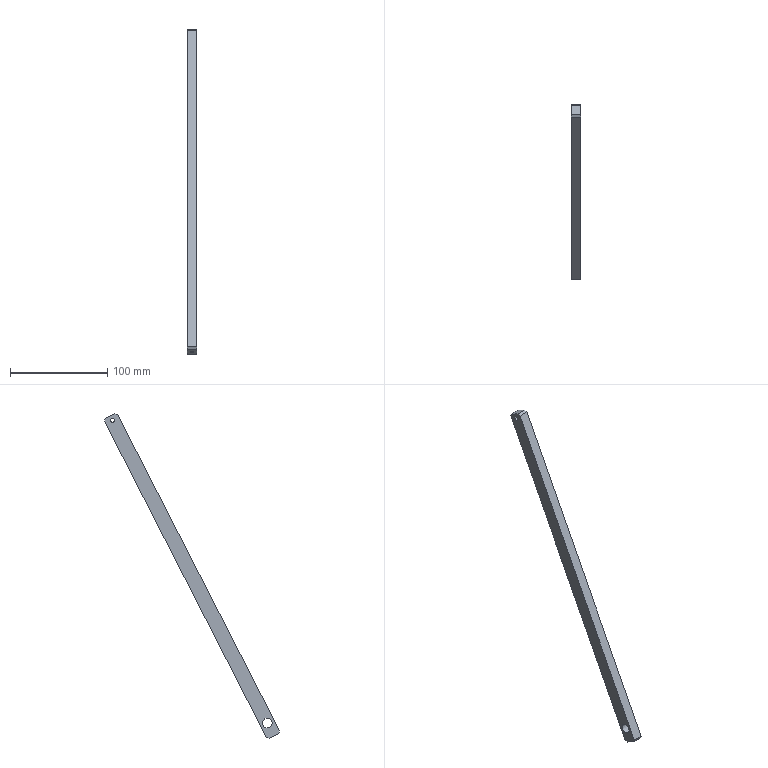Component | SolidWorks | ElectricalBoxAssembly2-1_SwingArm-1 | 1 solid | 16 faces | box 10 x 180.09 x 334.39 mm | volume 54356 mm3 | plane 10 | cylinder 6 | commonest cylinder face diameters 4.2 x4 10 x2
build123d program:
from build123d import *

# Parameters (mm, degrees)
SKETCH1_W             = 370
SKETCH1_H             = 15
SKETCH1_R             = 5
BOSS_EXTRUDE1_DEPTH   = 10
M5_TAPPED_HOLE1_D     = 4.2
M5_TAPPED_HOLE2_D     = 4.2
M5_TAPPED_HOLE2_DEPTH = 15
M5_TAPPED_HOLE2_TIP   = 1.262
CHAMFER1_SIZE         = 2


with BuildPart() as part:
    # Sketch1 → Boss-Extrude1 (new body)
    with BuildSketch(Plane.XY):
        Rectangle(SKETCH1_W, SKETCH1_H)
        with Locations((170, 0)):
            Circle(SKETCH1_R, mode=Mode.SUBTRACT)
    extrude(amount=BOSS_EXTRUDE1_DEPTH)

    # M5 Tapped Hole1 (through all)
    with Locations(Plane.XY.offset(10)):
        with Locations((-180, 0)):
            Hole(M5_TAPPED_HOLE1_D / 2)

    # M5 Tapped Hole2
    with Locations(Plane(origin=(185, 0, 0), x_dir=(0, 0, -1), z_dir=(1, 0, 0))):
        with Locations((-5, 0)):
            Hole(M5_TAPPED_HOLE2_D / 2, depth=M5_TAPPED_HOLE2_DEPTH)
            with Locations((0, 0, -(M5_TAPPED_HOLE2_DEPTH + M5_TAPPED_HOLE2_TIP / 2))):  # 118° drill point
                Cone(0, M5_TAPPED_HOLE2_D / 2, M5_TAPPED_HOLE2_TIP, mode=Mode.SUBTRACT)

    # Chamfer1
    chamfer1_edges = [part.edges().sort_by_distance(p)[0] for p in [
        (185, -7.5, 5),
        (-185, -7.5, 5),
        (-185, 7.5, 5),
        (185, 7.5, 5),
    ]]
    chamfer(chamfer1_edges, length=CHAMFER1_SIZE)


solid = part.part

# Placed as in the assembly
solid = solid.moved(Location((750.468, 292.11, 1827.734), (152.899, -90, 0)))
STEP:
#1=CARTESIAN_POINT('',(29.432,8.362,65.825));
#2=VERTEX_POINT('',#1);
#3=CARTESIAN_POINT('',(29.266,8.362,65.825));
#4=VERTEX_POINT('',#3);
#5=CARTESIAN_POINT('',(29.432,8.362,65.825));
#6=CARTESIAN_POINT('',(29.432,8.367,65.822));
#7=CARTESIAN_POINT('',(29.431,8.372,65.82));
#8=CARTESIAN_POINT('',(29.429,8.381,65.816));
#9=CARTESIAN_POINT('',(29.428,8.386,65.814));
#10=CARTESIAN_POINT('',(29.423,8.396,65.811));
#11=CARTESIAN_POINT('',(29.421,8.401,65.81));
#12=CARTESIAN_POINT('',(29.415,8.41,65.808));
#13=CARTESIAN_POINT('',(29.411,8.414,65.807));
#14=CARTESIAN_POINT('',(29.4,8.426,65.805));
#15=CARTESIAN_POINT('',(29.391,8.432,65.804));
#16=CARTESIAN_POINT('',(29.376,8.439,65.803));
#17=CARTESIAN_POINT('',(29.371,8.441,65.803));
#18=CARTESIAN_POINT('',(29.36,8.443,65.803));
#19=CARTESIAN_POINT('',(29.355,8.444,65.803));
#20=CARTESIAN_POINT('',(29.344,8.444,65.803));
#21=CARTESIAN_POINT('',(29.338,8.443,65.803));
#22=CARTESIAN_POINT('',(29.328,8.441,65.803));
#23=CARTESIAN_POINT('',(29.322,8.439,65.803));
#24=CARTESIAN_POINT('',(29.312,8.434,65.804));
#25=CARTESIAN_POINT('',(29.308,8.432,65.804));
#26=CARTESIAN_POINT('',(29.299,8.425,65.805));
#27=CARTESIAN_POINT('',(29.294,8.422,65.805));
#28=CARTESIAN_POINT('',(29.287,8.414,65.807));
#29=CARTESIAN_POINT('',(29.284,8.41,65.808));
#30=CARTESIAN_POINT('',(29.278,8.401,65.81));
#31=CARTESIAN_POINT('',(29.275,8.396,65.811));
#32=CARTESIAN_POINT('',(29.269,8.382,65.816));
#33=CARTESIAN_POINT('',(29.266,8.371,65.82));
#34=CARTESIAN_POINT('',(29.266,8.362,65.825));
#35=B_SPLINE_CURVE_WITH_KNOTS('',3,(#5,#6,#7,#8,#9,#10,#11,#12,#13,#14,#15,#16,#17,#18,#19,#20,#21,#22,#23,#24,#25,#26,#27,#28,#29,#30,#31,#32,#33,#34),.UNSPECIFIED.,.F.,.F.,(4,2,2,2,2,2,2,2,2,2,2,2,2,2,4),(0.,0.0004152,0.0008304,0.001246,0.001661,0.002491,0.002907,0.003322,0.003737,0.004152,0.004567,0.004983,0.005398,0.005813,0.006644),.UNSPECIFIED.);
#36=EDGE_CURVE('',#2,#4,#35,.T.);
#37=ORIENTED_EDGE('',*,*,#36,.T.);
#38=CARTESIAN_POINT('',(29.266,8.182,65.474));
#39=VERTEX_POINT('',#38);
#40=CARTESIAN_POINT('',(29.266,8.182,65.474));
#41=DIRECTION('',(0.,-0.4556,-0.8902));
#42=VECTOR('',#41,39.37);
#43=LINE('',#40,#42);
#44=EDGE_CURVE('',#4,#39,#43,.T.);
#45=ORIENTED_EDGE('',*,*,#44,.T.);
#46=CARTESIAN_POINT('',(29.432,8.182,65.474));
#47=VERTEX_POINT('',#46);
#48=CARTESIAN_POINT('',(29.349,8.182,65.474));
#49=DIRECTION('',(0.,-0.4556,-0.8902));
#50=DIRECTION('',(1.,0.,0.));
#51=AXIS2_PLACEMENT_3D('',#48,#49,#50);
#52=CIRCLE('',#51,0.08268);
#53=EDGE_CURVE('',#39,#47,#52,.T.);
#54=ORIENTED_EDGE('',*,*,#53,.T.);
#55=CARTESIAN_POINT('',(29.432,8.182,65.474));
#56=DIRECTION('',(0.,-0.4556,-0.8902));
#57=VECTOR('',#56,39.37);
#58=LINE('',#55,#57);
#59=EDGE_CURVE('',#2,#47,#58,.T.);
#60=ORIENTED_EDGE('',*,*,#59,.F.);
#61=EDGE_LOOP('',(#37,#45,#54,#60));
#62=FACE_OUTER_BOUND('',#61,.T.);
#63=CARTESIAN_POINT('',(29.349,8.182,65.474));
#64=DIRECTION('',(0.,-0.4556,-0.8902));
#65=DIRECTION('',(1.,0.,0.));
#66=AXIS2_PLACEMENT_3D('',#63,#64,#65);
#67=CYLINDRICAL_SURFACE('',#66,0.08268);
#68=ADVANCED_FACE('',(#62),#67,.F.);
#69=CARTESIAN_POINT('',(29.546,14.766,78.34));
#70=VERTEX_POINT('',#69);
#71=CARTESIAN_POINT('',(29.546,14.691,78.193));
#72=VERTEX_POINT('',#71);
#73=CARTESIAN_POINT('',(29.546,14.729,78.267));
#74=DIRECTION('',(-1.,0.,-0.));
#75=DIRECTION('',(0.,-0.4556,-0.8902));
#76=AXIS2_PLACEMENT_3D('',#73,#74,#75);
#77=CIRCLE('',#76,0.08268);
#78=EDGE_CURVE('',#70,#72,#77,.T.);
#79=ORIENTED_EDGE('',*,*,#78,.F.);
#80=CARTESIAN_POINT('',(29.152,14.766,78.34));
#81=VERTEX_POINT('',#80);
#82=CARTESIAN_POINT('',(29.152,14.766,78.34));
#83=DIRECTION('',(-1.,0.,-0.));
#84=VECTOR('',#83,39.37);
#85=LINE('',#82,#84);
#86=EDGE_CURVE('',#70,#81,#85,.T.);
#87=ORIENTED_EDGE('',*,*,#86,.T.);
#88=CARTESIAN_POINT('',(29.152,14.691,78.193));
#89=VERTEX_POINT('',#88);
#90=CARTESIAN_POINT('',(29.152,14.729,78.267));
#91=DIRECTION('',(-1.,0.,-0.));
#92=DIRECTION('',(0.,-0.4556,-0.8902));
#93=AXIS2_PLACEMENT_3D('',#90,#91,#92);
#94=CIRCLE('',#93,0.08268);
#95=EDGE_CURVE('',#81,#89,#94,.T.);
#96=ORIENTED_EDGE('',*,*,#95,.T.);
#97=CARTESIAN_POINT('',(29.152,14.691,78.193));
#98=DIRECTION('',(-1.,0.,-0.));
#99=VECTOR('',#98,39.37);
#100=LINE('',#97,#99);
#101=EDGE_CURVE('',#72,#89,#100,.T.);
#102=ORIENTED_EDGE('',*,*,#101,.F.);
#103=EDGE_LOOP('',(#79,#87,#96,#102));
#104=FACE_OUTER_BOUND('',#103,.T.);
#105=CARTESIAN_POINT('',(29.152,14.729,78.267));
#106=DIRECTION('',(-1.,0.,-0.));
#107=DIRECTION('',(0.,-0.4556,-0.8902));
#108=AXIS2_PLACEMENT_3D('',#105,#106,#107);
#109=CYLINDRICAL_SURFACE('',#108,0.08268);
#110=ADVANCED_FACE('',(#104),#109,.F.);
#111=CARTESIAN_POINT('',(29.152,8.541,66.175));
#112=VERTEX_POINT('',#111);
#113=CARTESIAN_POINT('',(29.152,8.362,65.825));
#114=VERTEX_POINT('',#113);
#115=CARTESIAN_POINT('',(29.152,8.451,66.));
#116=DIRECTION('',(-1.,0.,-0.));
#117=DIRECTION('',(0.,-0.4556,-0.8902));
#118=AXIS2_PLACEMENT_3D('',#115,#116,#117);
#119=CIRCLE('',#118,0.1969);
#120=EDGE_CURVE('',#112,#114,#119,.T.);
#121=ORIENTED_EDGE('',*,*,#120,.T.);
#122=CARTESIAN_POINT('',(29.152,8.362,65.825));
#123=DIRECTION('',(1.,0.,0.));
#124=VECTOR('',#123,39.37);
#125=LINE('',#122,#124);
#126=EDGE_CURVE('',#114,#4,#125,.T.);
#127=ORIENTED_EDGE('',*,*,#126,.T.);
#128=ORIENTED_EDGE('',*,*,#36,.F.);
#129=CARTESIAN_POINT('',(29.546,8.362,65.825));
#130=VERTEX_POINT('',#129);
#131=CARTESIAN_POINT('',(29.152,8.362,65.825));
#132=DIRECTION('',(1.,0.,0.));
#133=VECTOR('',#132,39.37);
#134=LINE('',#131,#133);
#135=EDGE_CURVE('',#2,#130,#134,.T.);
#136=ORIENTED_EDGE('',*,*,#135,.T.);
#137=CARTESIAN_POINT('',(29.546,8.541,66.175));
#138=VERTEX_POINT('',#137);
#139=CARTESIAN_POINT('',(29.546,8.451,66.));
#140=DIRECTION('',(-1.,0.,-0.));
#141=DIRECTION('',(0.,-0.4556,-0.8902));
#142=AXIS2_PLACEMENT_3D('',#139,#140,#141);
#143=CIRCLE('',#142,0.1969);
#144=EDGE_CURVE('',#138,#130,#143,.T.);
#145=ORIENTED_EDGE('',*,*,#144,.F.);
#146=CARTESIAN_POINT('',(29.152,8.541,66.175));
#147=DIRECTION('',(1.,0.,0.));
#148=VECTOR('',#147,39.37);
#149=LINE('',#146,#148);
#150=EDGE_CURVE('',#112,#138,#149,.T.);
#151=ORIENTED_EDGE('',*,*,#150,.F.);
#152=EDGE_LOOP('',(#121,#127,#128,#136,#145,#151));
#153=FACE_OUTER_BOUND('',#152,.T.);
#154=CARTESIAN_POINT('',(29.152,8.451,66.));
#155=DIRECTION('',(1.,0.,0.));
#156=DIRECTION('',(0.,0.4556,0.8902));
#157=AXIS2_PLACEMENT_3D('',#154,#155,#156);
#158=CYLINDRICAL_SURFACE('',#157,0.1969);
#159=ADVANCED_FACE('',(#153),#158,.F.);
#160=CARTESIAN_POINT('',(29.152,14.729,78.267));
#161=DIRECTION('',(-1.,0.,-0.));
#162=DIRECTION('',(0.,-0.4556,-0.8902));
#163=AXIS2_PLACEMENT_3D('',#160,#161,#162);
#164=CIRCLE('',#163,0.08268);
#165=EDGE_CURVE('',#89,#81,#164,.T.);
#166=ORIENTED_EDGE('',*,*,#165,.F.);
#167=ORIENTED_EDGE('',*,*,#95,.F.);
#168=EDGE_LOOP('',(#166,#167));
#169=FACE_BOUND('',#168,.T.);
#170=CARTESIAN_POINT('',(29.152,15.045,78.237));
#171=VERTEX_POINT('',#170);
#172=CARTESIAN_POINT('',(29.152,8.481,65.41));
#173=VERTEX_POINT('',#172);
#174=CARTESIAN_POINT('',(29.152,15.081,78.307));
#175=DIRECTION('',(0.,-0.4556,-0.8902));
#176=VECTOR('',#175,39.37);
#177=LINE('',#174,#176);
#178=EDGE_CURVE('',#171,#173,#177,.T.);
#179=ORIENTED_EDGE('',*,*,#178,.T.);
#180=CARTESIAN_POINT('',(29.152,8.375,65.376));
#181=VERTEX_POINT('',#180);
#182=CARTESIAN_POINT('',(29.152,13.13,66.911));
#183=DIRECTION('',(0.,-0.9516,-0.3073));
#184=VECTOR('',#183,39.37);
#185=LINE('',#182,#184);
#186=EDGE_CURVE('',#173,#181,#185,.T.);
#187=ORIENTED_EDGE('',*,*,#186,.T.);
#188=CARTESIAN_POINT('',(29.152,7.99,65.573));
#189=VERTEX_POINT('',#188);
#190=CARTESIAN_POINT('',(29.152,7.92,65.609));
#191=DIRECTION('',(-0.,-0.8902,0.4556));
#192=VECTOR('',#191,39.37);
#193=LINE('',#190,#192);
#194=EDGE_CURVE('',#181,#189,#193,.T.);
#195=ORIENTED_EDGE('',*,*,#194,.T.);
#196=CARTESIAN_POINT('',(29.152,7.955,65.679));
#197=VERTEX_POINT('',#196);
#198=CARTESIAN_POINT('',(29.152,6.454,70.328));
#199=DIRECTION('',(-0.,-0.3073,0.9516));
#200=VECTOR('',#199,39.37);
#201=LINE('',#198,#200);
#202=EDGE_CURVE('',#189,#197,#201,.T.);
#203=ORIENTED_EDGE('',*,*,#202,.T.);
#204=CARTESIAN_POINT('',(29.152,14.52,78.506));
#205=VERTEX_POINT('',#204);
#206=CARTESIAN_POINT('',(29.152,14.556,78.576));
#207=DIRECTION('',(-0.,0.4556,0.8902));
#208=VECTOR('',#207,39.37);
#209=LINE('',#206,#208);
#210=EDGE_CURVE('',#197,#205,#209,.T.);
#211=ORIENTED_EDGE('',*,*,#210,.T.);
#212=CARTESIAN_POINT('',(29.152,14.626,78.54));
#213=VERTEX_POINT('',#212);
#214=CARTESIAN_POINT('',(29.152,9.87,77.005));
#215=DIRECTION('',(-0.,0.9516,0.3073));
#216=VECTOR('',#215,39.37);
#217=LINE('',#214,#216);
#218=EDGE_CURVE('',#205,#213,#217,.T.);
#219=ORIENTED_EDGE('',*,*,#218,.T.);
#220=CARTESIAN_POINT('',(29.152,15.011,78.343));
#221=VERTEX_POINT('',#220);
#222=CARTESIAN_POINT('',(29.152,14.556,78.576));
#223=DIRECTION('',(0.,0.8902,-0.4556));
#224=VECTOR('',#223,39.37);
#225=LINE('',#222,#224);
#226=EDGE_CURVE('',#213,#221,#225,.T.);
#227=ORIENTED_EDGE('',*,*,#226,.T.);
#228=CARTESIAN_POINT('',(29.152,16.547,73.588));
#229=DIRECTION('',(0.,0.3073,-0.9516));
#230=VECTOR('',#229,39.37);
#231=LINE('',#228,#230);
#232=EDGE_CURVE('',#221,#171,#231,.T.);
#233=ORIENTED_EDGE('',*,*,#232,.T.);
#234=EDGE_LOOP('',(#179,#187,#195,#203,#211,#219,#227,#233));
#235=FACE_OUTER_BOUND('',#234,.T.);
#236=ORIENTED_EDGE('',*,*,#120,.F.);
#237=CARTESIAN_POINT('',(29.152,8.451,66.));
#238=DIRECTION('',(-1.,0.,-0.));
#239=DIRECTION('',(0.,-0.4556,-0.8902));
#240=AXIS2_PLACEMENT_3D('',#237,#238,#239);
#241=CIRCLE('',#240,0.1969);
#242=EDGE_CURVE('',#114,#112,#241,.T.);
#243=ORIENTED_EDGE('',*,*,#242,.F.);
#244=EDGE_LOOP('',(#236,#243));
#245=FACE_BOUND('',#244,.T.);
#246=CARTESIAN_POINT('',(29.152,11.5,71.958));
#247=DIRECTION('',(-1.,-0.,-0.));
#248=DIRECTION('',(0.,-0.4556,-0.8902));
#249=AXIS2_PLACEMENT_3D('',#246,#247,#248);
#250=PLANE('',#249);
#251=ADVANCED_FACE('',(#169,#235,#245),#250,.T.);
#252=CARTESIAN_POINT('',(29.546,14.729,78.267));
#253=DIRECTION('',(-1.,0.,-0.));
#254=DIRECTION('',(0.,-0.4556,-0.8902));
#255=AXIS2_PLACEMENT_3D('',#252,#253,#254);
#256=CIRCLE('',#255,0.08268);
#257=EDGE_CURVE('',#72,#70,#256,.T.);
#258=ORIENTED_EDGE('',*,*,#257,.T.);
#259=ORIENTED_EDGE('',*,*,#78,.T.);
#260=EDGE_LOOP('',(#258,#259));
#261=FACE_BOUND('',#260,.T.);
#262=CARTESIAN_POINT('',(29.546,8.375,65.376));
#263=VERTEX_POINT('',#262);
#264=CARTESIAN_POINT('',(29.546,7.99,65.573));
#265=VERTEX_POINT('',#264);
#266=CARTESIAN_POINT('',(29.546,7.92,65.609));
#267=DIRECTION('',(-0.,-0.8902,0.4556));
#268=VECTOR('',#267,39.37);
#269=LINE('',#266,#268);
#270=EDGE_CURVE('',#263,#265,#269,.T.);
#271=ORIENTED_EDGE('',*,*,#270,.F.);
#272=CARTESIAN_POINT('',(29.546,8.481,65.41));
#273=VERTEX_POINT('',#272);
#274=CARTESIAN_POINT('',(29.546,8.375,65.376));
#275=DIRECTION('',(-0.,0.9516,0.3073));
#276=VECTOR('',#275,39.37);
#277=LINE('',#274,#276);
#278=EDGE_CURVE('',#263,#273,#277,.T.);
#279=ORIENTED_EDGE('',*,*,#278,.T.);
#280=CARTESIAN_POINT('',(29.546,15.045,78.237));
#281=VERTEX_POINT('',#280);
#282=CARTESIAN_POINT('',(29.546,15.081,78.307));
#283=DIRECTION('',(0.,-0.4556,-0.8902));
#284=VECTOR('',#283,39.37);
#285=LINE('',#282,#284);
#286=EDGE_CURVE('',#281,#273,#285,.T.);
#287=ORIENTED_EDGE('',*,*,#286,.F.);
#288=CARTESIAN_POINT('',(29.546,15.011,78.343));
#289=VERTEX_POINT('',#288);
#290=CARTESIAN_POINT('',(29.546,15.045,78.237));
#291=DIRECTION('',(-0.,-0.3073,0.9516));
#292=VECTOR('',#291,39.37);
#293=LINE('',#290,#292);
#294=EDGE_CURVE('',#281,#289,#293,.T.);
#295=ORIENTED_EDGE('',*,*,#294,.T.);
#296=CARTESIAN_POINT('',(29.546,14.626,78.54));
#297=VERTEX_POINT('',#296);
#298=CARTESIAN_POINT('',(29.546,14.556,78.576));
#299=DIRECTION('',(0.,0.8902,-0.4556));
#300=VECTOR('',#299,39.37);
#301=LINE('',#298,#300);
#302=EDGE_CURVE('',#297,#289,#301,.T.);
#303=ORIENTED_EDGE('',*,*,#302,.F.);
#304=CARTESIAN_POINT('',(29.546,14.52,78.506));
#305=VERTEX_POINT('',#304);
#306=CARTESIAN_POINT('',(29.546,14.626,78.54));
#307=DIRECTION('',(0.,-0.9516,-0.3073));
#308=VECTOR('',#307,39.37);
#309=LINE('',#306,#308);
#310=EDGE_CURVE('',#297,#305,#309,.T.);
#311=ORIENTED_EDGE('',*,*,#310,.T.);
#312=CARTESIAN_POINT('',(29.546,7.955,65.679));
#313=VERTEX_POINT('',#312);
#314=CARTESIAN_POINT('',(29.546,14.556,78.576));
#315=DIRECTION('',(-0.,0.4556,0.8902));
#316=VECTOR('',#315,39.37);
#317=LINE('',#314,#316);
#318=EDGE_CURVE('',#313,#305,#317,.T.);
#319=ORIENTED_EDGE('',*,*,#318,.F.);
#320=CARTESIAN_POINT('',(29.546,7.955,65.679));
#321=DIRECTION('',(0.,0.3073,-0.9516));
#322=VECTOR('',#321,39.37);
#323=LINE('',#320,#322);
#324=EDGE_CURVE('',#313,#265,#323,.T.);
#325=ORIENTED_EDGE('',*,*,#324,.T.);
#326=EDGE_LOOP('',(#271,#279,#287,#295,#303,#311,#319,#325));
#327=FACE_OUTER_BOUND('',#326,.T.);
#328=ORIENTED_EDGE('',*,*,#144,.T.);
#329=CARTESIAN_POINT('',(29.546,8.451,66.));
#330=DIRECTION('',(-1.,0.,-0.));
#331=DIRECTION('',(0.,-0.4556,-0.8902));
#332=AXIS2_PLACEMENT_3D('',#329,#330,#331);
#333=CIRCLE('',#332,0.1969);
#334=EDGE_CURVE('',#130,#138,#333,.T.);
#335=ORIENTED_EDGE('',*,*,#334,.T.);
#336=EDGE_LOOP('',(#328,#335));
#337=FACE_BOUND('',#336,.T.);
#338=CARTESIAN_POINT('',(29.546,11.5,71.958));
#339=DIRECTION('',(-1.,-0.,-0.));
#340=DIRECTION('',(0.,-0.4556,-0.8902));
#341=AXIS2_PLACEMENT_3D('',#338,#339,#340);
#342=PLANE('',#341);
#343=ADVANCED_FACE('',(#261,#327,#337),#342,.F.);
#344=CARTESIAN_POINT('',(29.349,8.182,65.474));
#345=DIRECTION('',(0.,-0.4556,-0.8902));
#346=DIRECTION('',(1.,0.,0.));
#347=AXIS2_PLACEMENT_3D('',#344,#345,#346);
#348=CIRCLE('',#347,0.08268);
#349=EDGE_CURVE('',#47,#39,#348,.T.);
#350=ORIENTED_EDGE('',*,*,#349,.F.);
#351=ORIENTED_EDGE('',*,*,#53,.F.);
#352=EDGE_LOOP('',(#350,#351));
#353=FACE_BOUND('',#352,.T.);
#354=ORIENTED_EDGE('',*,*,#194,.F.);
#355=CARTESIAN_POINT('',(29.152,8.375,65.376));
#356=DIRECTION('',(1.,0.,0.));
#357=VECTOR('',#356,39.37);
#358=LINE('',#355,#357);
#359=EDGE_CURVE('',#181,#263,#358,.T.);
#360=ORIENTED_EDGE('',*,*,#359,.T.);
#361=ORIENTED_EDGE('',*,*,#270,.T.);
#362=CARTESIAN_POINT('',(29.152,7.99,65.573));
#363=DIRECTION('',(-1.,0.,-0.));
#364=VECTOR('',#363,39.37);
#365=LINE('',#362,#364);
#366=EDGE_CURVE('',#265,#189,#365,.T.);
#367=ORIENTED_EDGE('',*,*,#366,.T.);
#368=EDGE_LOOP('',(#354,#360,#361,#367));
#369=FACE_OUTER_BOUND('',#368,.T.);
#370=CARTESIAN_POINT('',(29.152,7.92,65.609));
#371=DIRECTION('',(-0.,0.4556,0.8902));
#372=DIRECTION('',(-1.,0.,-0.));
#373=AXIS2_PLACEMENT_3D('',#370,#371,#372);
#374=PLANE('',#373);
#375=ADVANCED_FACE('',(#353,#369),#374,.F.);
#376=ORIENTED_EDGE('',*,*,#210,.F.);
#377=CARTESIAN_POINT('',(29.152,7.955,65.679));
#378=DIRECTION('',(1.,0.,0.));
#379=VECTOR('',#378,39.37);
#380=LINE('',#377,#379);
#381=EDGE_CURVE('',#197,#313,#380,.T.);
#382=ORIENTED_EDGE('',*,*,#381,.T.);
#383=ORIENTED_EDGE('',*,*,#318,.T.);
#384=CARTESIAN_POINT('',(29.152,14.52,78.506));
#385=DIRECTION('',(-1.,0.,-0.));
#386=VECTOR('',#385,39.37);
#387=LINE('',#384,#386);
#388=EDGE_CURVE('',#305,#205,#387,.T.);
#389=ORIENTED_EDGE('',*,*,#388,.T.);
#390=EDGE_LOOP('',(#376,#382,#383,#389));
#391=FACE_OUTER_BOUND('',#390,.T.);
#392=CARTESIAN_POINT('',(29.152,14.556,78.576));
#393=DIRECTION('',(0.,0.8902,-0.4556));
#394=DIRECTION('',(1.,0.,0.));
#395=AXIS2_PLACEMENT_3D('',#392,#393,#394);
#396=PLANE('',#395);
#397=ADVANCED_FACE('',(#391),#396,.F.);
#398=ORIENTED_EDGE('',*,*,#302,.T.);
#399=CARTESIAN_POINT('',(29.152,15.011,78.343));
#400=DIRECTION('',(-1.,0.,-0.));
#401=VECTOR('',#400,39.37);
#402=LINE('',#399,#401);
#403=EDGE_CURVE('',#289,#221,#402,.T.);
#404=ORIENTED_EDGE('',*,*,#403,.T.);
#405=ORIENTED_EDGE('',*,*,#226,.F.);
#406=CARTESIAN_POINT('',(29.152,14.626,78.54));
#407=DIRECTION('',(1.,0.,0.));
#408=VECTOR('',#407,39.37);
#409=LINE('',#406,#408);
#410=EDGE_CURVE('',#213,#297,#409,.T.);
#411=ORIENTED_EDGE('',*,*,#410,.T.);
#412=EDGE_LOOP('',(#398,#404,#405,#411));
#413=FACE_OUTER_BOUND('',#412,.T.);
#414=CARTESIAN_POINT('',(29.152,14.556,78.576));
#415=DIRECTION('',(0.,-0.4556,-0.8902));
#416=DIRECTION('',(1.,0.,0.));
#417=AXIS2_PLACEMENT_3D('',#414,#415,#416);
#418=PLANE('',#417);
#419=ADVANCED_FACE('',(#413),#418,.F.);
#420=ORIENTED_EDGE('',*,*,#286,.T.);
#421=CARTESIAN_POINT('',(29.152,8.481,65.41));
#422=DIRECTION('',(-1.,0.,-0.));
#423=VECTOR('',#422,39.37);
#424=LINE('',#421,#423);
#425=EDGE_CURVE('',#273,#173,#424,.T.);
#426=ORIENTED_EDGE('',*,*,#425,.T.);
#427=ORIENTED_EDGE('',*,*,#178,.F.);
#428=CARTESIAN_POINT('',(29.152,15.045,78.237));
#429=DIRECTION('',(1.,0.,0.));
#430=VECTOR('',#429,39.37);
#431=LINE('',#428,#430);
#432=EDGE_CURVE('',#171,#281,#431,.T.);
#433=ORIENTED_EDGE('',*,*,#432,.T.);
#434=EDGE_LOOP('',(#420,#426,#427,#433));
#435=FACE_OUTER_BOUND('',#434,.T.);
#436=CARTESIAN_POINT('',(29.152,15.081,78.307));
#437=DIRECTION('',(-0.,-0.8902,0.4556));
#438=DIRECTION('',(-1.,0.,-0.));
#439=AXIS2_PLACEMENT_3D('',#436,#437,#438);
#440=PLANE('',#439);
#441=ADVANCED_FACE('',(#435),#440,.F.);
#442=ORIENTED_EDGE('',*,*,#126,.F.);
#443=ORIENTED_EDGE('',*,*,#242,.T.);
#444=ORIENTED_EDGE('',*,*,#150,.T.);
#445=ORIENTED_EDGE('',*,*,#334,.F.);
#446=ORIENTED_EDGE('',*,*,#135,.F.);
#447=CARTESIAN_POINT('',(29.266,8.362,65.825));
#448=CARTESIAN_POINT('',(29.266,8.357,65.827));
#449=CARTESIAN_POINT('',(29.267,8.352,65.83));
#450=CARTESIAN_POINT('',(29.269,8.343,65.836));
#451=CARTESIAN_POINT('',(29.271,8.339,65.839));
#452=CARTESIAN_POINT('',(29.275,8.33,65.845));
#453=CARTESIAN_POINT('',(29.278,8.327,65.848));
#454=CARTESIAN_POINT('',(29.284,8.32,65.854));
#455=CARTESIAN_POINT('',(29.287,8.317,65.857));
#456=CARTESIAN_POINT('',(29.295,8.311,65.862));
#457=CARTESIAN_POINT('',(29.299,8.308,65.865));
#458=CARTESIAN_POINT('',(29.308,8.304,65.869));
#459=CARTESIAN_POINT('',(29.312,8.302,65.871));
#460=CARTESIAN_POINT('',(29.322,8.299,65.875));
#461=CARTESIAN_POINT('',(29.327,8.298,65.876));
#462=CARTESIAN_POINT('',(29.338,8.297,65.878));
#463=CARTESIAN_POINT('',(29.344,8.296,65.879));
#464=CARTESIAN_POINT('',(29.36,8.296,65.879));
#465=CARTESIAN_POINT('',(29.371,8.298,65.877));
#466=CARTESIAN_POINT('',(29.386,8.302,65.871));
#467=CARTESIAN_POINT('',(29.391,8.304,65.869));
#468=CARTESIAN_POINT('',(29.4,8.308,65.865));
#469=CARTESIAN_POINT('',(29.404,8.311,65.862));
#470=CARTESIAN_POINT('',(29.411,8.317,65.856));
#471=CARTESIAN_POINT('',(29.415,8.32,65.854));
#472=CARTESIAN_POINT('',(29.421,8.327,65.848));
#473=CARTESIAN_POINT('',(29.423,8.33,65.845));
#474=CARTESIAN_POINT('',(29.428,8.339,65.839));
#475=CARTESIAN_POINT('',(29.429,8.343,65.836));
#476=CARTESIAN_POINT('',(29.431,8.352,65.83));
#477=CARTESIAN_POINT('',(29.432,8.357,65.827));
#478=CARTESIAN_POINT('',(29.432,8.362,65.825));
#479=B_SPLINE_CURVE_WITH_KNOTS('',3,(#447,#448,#449,#450,#451,#452,#453,#454,#455,#456,#457,#458,#459,#460,#461,#462,#463,#464,#465,#466,#467,#468,#469,#470,#471,#472,#473,#474,#475,#476,#477,#478),.UNSPECIFIED.,.F.,.F.,(4,2,2,2,2,2,2,2,2,2,2,2,2,2,2,4),(0.006644,0.007058,0.007473,0.007888,0.008303,0.008718,0.009133,0.009548,0.009963,0.01079,0.01121,0.01162,0.01204,0.01245,0.01287,0.01328),.UNSPECIFIED.);
#480=EDGE_CURVE('',#4,#2,#479,.T.);
#481=ORIENTED_EDGE('',*,*,#480,.F.);
#482=EDGE_LOOP('',(#442,#443,#444,#445,#446,#481));
#483=FACE_OUTER_BOUND('',#482,.T.);
#484=CARTESIAN_POINT('',(29.152,8.451,66.));
#485=DIRECTION('',(1.,0.,0.));
#486=DIRECTION('',(0.,0.4556,0.8902));
#487=AXIS2_PLACEMENT_3D('',#484,#485,#486);
#488=CYLINDRICAL_SURFACE('',#487,0.1969);
#489=ADVANCED_FACE('',(#483),#488,.F.);
#490=ORIENTED_EDGE('',*,*,#86,.F.);
#491=ORIENTED_EDGE('',*,*,#257,.F.);
#492=ORIENTED_EDGE('',*,*,#101,.T.);
#493=ORIENTED_EDGE('',*,*,#165,.T.);
#494=EDGE_LOOP('',(#490,#491,#492,#493));
#495=FACE_OUTER_BOUND('',#494,.T.);
#496=CARTESIAN_POINT('',(29.152,14.729,78.267));
#497=DIRECTION('',(-1.,0.,-0.));
#498=DIRECTION('',(0.,-0.4556,-0.8902));
#499=AXIS2_PLACEMENT_3D('',#496,#497,#498);
#500=CYLINDRICAL_SURFACE('',#499,0.08268);
#501=ADVANCED_FACE('',(#495),#500,.F.);
#502=ORIENTED_EDGE('',*,*,#44,.F.);
#503=ORIENTED_EDGE('',*,*,#480,.T.);
#504=ORIENTED_EDGE('',*,*,#59,.T.);
#505=ORIENTED_EDGE('',*,*,#349,.T.);
#506=EDGE_LOOP('',(#502,#503,#504,#505));
#507=FACE_OUTER_BOUND('',#506,.T.);
#508=CARTESIAN_POINT('',(29.349,8.182,65.474));
#509=DIRECTION('',(0.,-0.4556,-0.8902));
#510=DIRECTION('',(1.,0.,0.));
#511=AXIS2_PLACEMENT_3D('',#508,#509,#510);
#512=CYLINDRICAL_SURFACE('',#511,0.08268);
#513=ADVANCED_FACE('',(#507),#512,.F.);
#514=ORIENTED_EDGE('',*,*,#186,.F.);
#515=ORIENTED_EDGE('',*,*,#425,.F.);
#516=ORIENTED_EDGE('',*,*,#278,.F.);
#517=ORIENTED_EDGE('',*,*,#359,.F.);
#518=EDGE_LOOP('',(#514,#515,#516,#517));
#519=FACE_OUTER_BOUND('',#518,.T.);
#520=CARTESIAN_POINT('',(29.152,8.375,65.376));
#521=DIRECTION('',(-0.,-0.3073,0.9516));
#522=DIRECTION('',(1.,0.,0.));
#523=AXIS2_PLACEMENT_3D('',#520,#521,#522);
#524=PLANE('',#523);
#525=ADVANCED_FACE('',(#519),#524,.F.);
#526=ORIENTED_EDGE('',*,*,#202,.F.);
#527=ORIENTED_EDGE('',*,*,#366,.F.);
#528=ORIENTED_EDGE('',*,*,#324,.F.);
#529=ORIENTED_EDGE('',*,*,#381,.F.);
#530=EDGE_LOOP('',(#526,#527,#528,#529));
#531=FACE_OUTER_BOUND('',#530,.T.);
#532=CARTESIAN_POINT('',(29.152,7.955,65.679));
#533=DIRECTION('',(-0.,0.9516,0.3073));
#534=DIRECTION('',(1.,0.,0.));
#535=AXIS2_PLACEMENT_3D('',#532,#533,#534);
#536=PLANE('',#535);
#537=ADVANCED_FACE('',(#531),#536,.F.);
#538=ORIENTED_EDGE('',*,*,#232,.F.);
#539=ORIENTED_EDGE('',*,*,#403,.F.);
#540=ORIENTED_EDGE('',*,*,#294,.F.);
#541=ORIENTED_EDGE('',*,*,#432,.F.);
#542=EDGE_LOOP('',(#538,#539,#540,#541));
#543=FACE_OUTER_BOUND('',#542,.T.);
#544=CARTESIAN_POINT('',(29.152,15.045,78.237));
#545=DIRECTION('',(0.,-0.9516,-0.3073));
#546=DIRECTION('',(1.,0.,0.));
#547=AXIS2_PLACEMENT_3D('',#544,#545,#546);
#548=PLANE('',#547);
#549=ADVANCED_FACE('',(#543),#548,.F.);
#550=ORIENTED_EDGE('',*,*,#218,.F.);
#551=ORIENTED_EDGE('',*,*,#388,.F.);
#552=ORIENTED_EDGE('',*,*,#310,.F.);
#553=ORIENTED_EDGE('',*,*,#410,.F.);
#554=EDGE_LOOP('',(#550,#551,#552,#553));
#555=FACE_OUTER_BOUND('',#554,.T.);
#556=CARTESIAN_POINT('',(29.152,14.626,78.54));
#557=DIRECTION('',(0.,0.3073,-0.9516));
#558=DIRECTION('',(1.,0.,0.));
#559=AXIS2_PLACEMENT_3D('',#556,#557,#558);
#560=PLANE('',#559);
#561=ADVANCED_FACE('',(#555),#560,.F.);
#562=CLOSED_SHELL('',(#68,#110,#159,#251,#343,#375,#397,#419,#441,#489,#501,#513,#525,#537,#549,#561));
#563=MANIFOLD_SOLID_BREP('',#562);
#564=CARTESIAN_POINT('',(0.,0.,0.));
#565=DIRECTION('',(0.,0.,1.));
#566=DIRECTION('',(1.,0.,0.));
#567=AXIS2_PLACEMENT_3D('',#564,#565,#566);
#568=(LENGTH_UNIT()NAMED_UNIT(*)SI_UNIT($,.METRE.));
#569=LENGTH_MEASURE_WITH_UNIT(LENGTH_MEASURE(0.0254),#568);
#570=DIMENSIONAL_EXPONENTS(1.,0.,0.,0.,0.,0.,0.);
#571=(CONVERSION_BASED_UNIT('',#569)LENGTH_UNIT()NAMED_UNIT(#570));
#572=UNCERTAINTY_MEASURE_WITH_UNIT(LENGTH_MEASURE(0.00001),#571,'','');
#573=(NAMED_UNIT(*)PLANE_ANGLE_UNIT()SI_UNIT($,.RADIAN.));
#574=(NAMED_UNIT(*)SI_UNIT($,.STERADIAN.)SOLID_ANGLE_UNIT());
#575=(GEOMETRIC_REPRESENTATION_CONTEXT(3)GLOBAL_UNCERTAINTY_ASSIGNED_CONTEXT((#572))GLOBAL_UNIT_ASSIGNED_CONTEXT((#571,#573,#574))REPRESENTATION_CONTEXT('',''));
#576=ADVANCED_BREP_SHAPE_REPRESENTATION('',(#563,#567),#575);
#577=COLOUR_RGB('',0.7922,0.8196,0.9333);
#578=FILL_AREA_STYLE_COLOUR('',#577);
#579=FILL_AREA_STYLE('',(#578));
#580=SURFACE_STYLE_FILL_AREA(#579);
#581=SURFACE_SIDE_STYLE('',(#580));
#582=SURFACE_STYLE_USAGE(.BOTH.,#581);
#583=PRESENTATION_STYLE_ASSIGNMENT((#582));
#584=STYLED_ITEM('',(#583),#563);
#585=(LENGTH_UNIT()NAMED_UNIT(*)SI_UNIT($,.METRE.));
#586=LENGTH_MEASURE_WITH_UNIT(LENGTH_MEASURE(0.0254),#585);
#587=DIMENSIONAL_EXPONENTS(1.,0.,0.,0.,0.,0.,0.);
#588=(CONVERSION_BASED_UNIT('',#586)LENGTH_UNIT()NAMED_UNIT(#587));
#589=UNCERTAINTY_MEASURE_WITH_UNIT(LENGTH_MEASURE(0.00001),#588,'','');
#590=(NAMED_UNIT(*)PLANE_ANGLE_UNIT()SI_UNIT($,.RADIAN.));
#591=(NAMED_UNIT(*)SI_UNIT($,.STERADIAN.)SOLID_ANGLE_UNIT());
#592=(GEOMETRIC_REPRESENTATION_CONTEXT(3)GLOBAL_UNCERTAINTY_ASSIGNED_CONTEXT((#589))GLOBAL_UNIT_ASSIGNED_CONTEXT((#588,#590,#591))REPRESENTATION_CONTEXT('',''));
#593=MECHANICAL_DESIGN_GEOMETRIC_PRESENTATION_REPRESENTATION('',(#584),#592);
#594=PRESENTATION_LAYER_ASSIGNMENT('','',(#584));